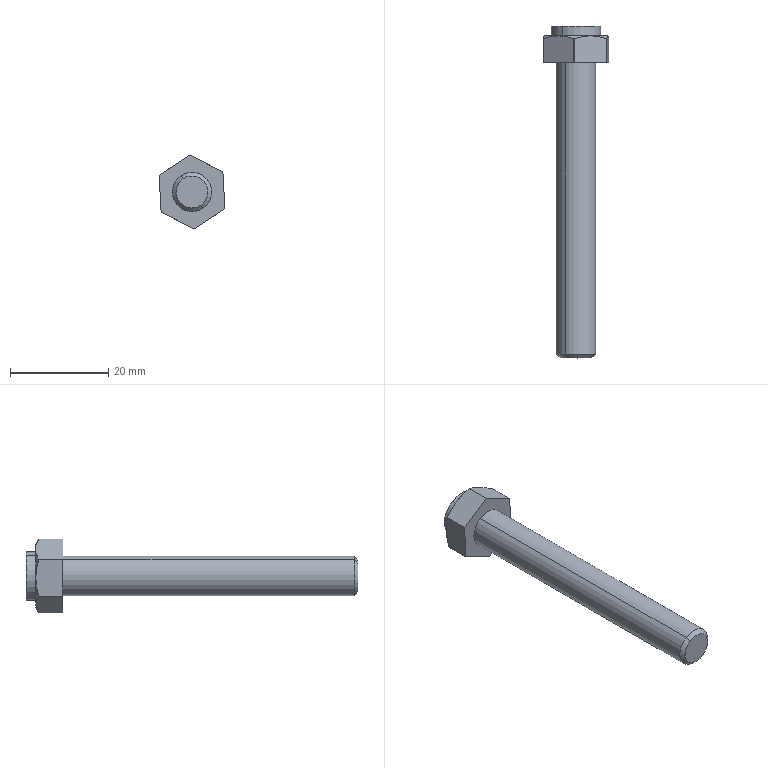Component | SolidWorks | UST8_60-1_UST8_60b-1 | 1 solid | 26 faces | box 13.39 x 67.5 x 14.98 mm | volume 3968 mm3 | plane 10 | cone 8 | cylinder 8 | commonest cylinder face diameters 15 x4 8 x2 10 x2
build123d program:
from build123d import *

# Parameters (mm, degrees)
SKETCH2_W          = 30
SKETCH2_H          = 30
CUT_EXTRUDE1_DEPTH = 7.5


with BuildPart() as part:
    # Sketch1 → Rotate1 (revolve)
    with BuildSketch(Plane.XY, mode=Mode.PRIVATE) as rotate1_sk:
        Polygon((-7.5, 0), (-7.5, 5), (-5.5, 5), (-5.5, 6.5), (-4.923, 7.5), (0, 7.5), (0, 4), (59.233, 4), (60, 3.233), (60, 0), align=None)
    revolve(rotate1_sk.sketch.rotate(Axis((60, 0, 0), (-1, 0, 0)), 270), axis=Axis((60, 0, 0), (-1, 0, 0)))

    # Sketch2 → Cut-Extrude1 (cut)
    with BuildSketch(Plane(origin=(0, 0, 0), x_dir=(0, 0, -1), z_dir=(1, 0, 0))):
        Rectangle(SKETCH2_W, SKETCH2_H)
        Polygon((-6.5, 3.753), (-6.5, -3.753), (0, -7.5), (6.5, -3.753), (6.5, 3.753), (0, 7.5), align=None, mode=Mode.SUBTRACT)
    extrude(amount=-CUT_EXTRUDE1_DEPTH, mode=Mode.SUBTRACT)


solid = part.part

# Placed as in the assembly
solid = solid.moved(Location((-861.708, 64.408, 89.188), (180, 33.156, 90)))